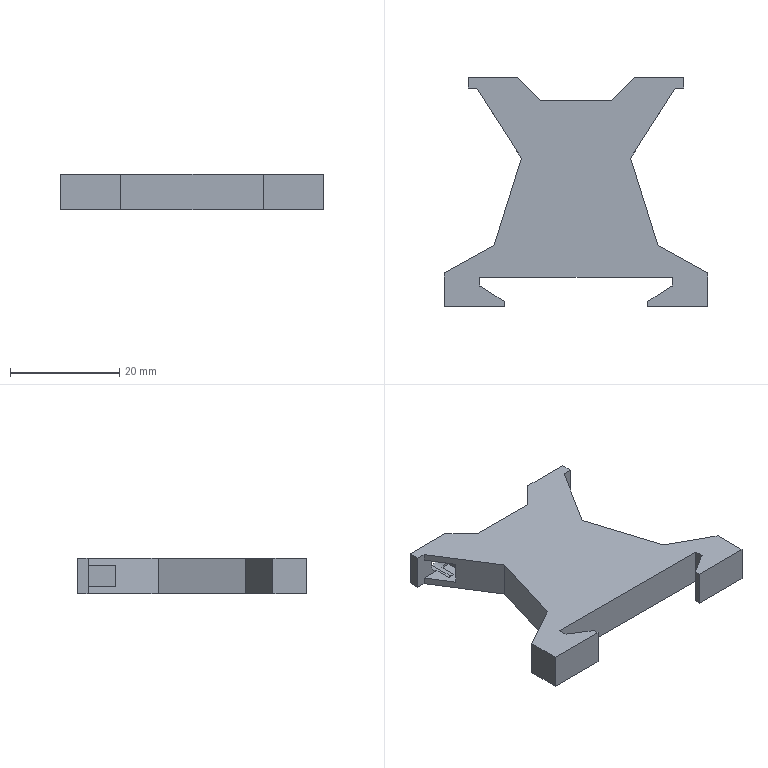Component | SolidWorks | UK5NVoltageTerminalBlock-12 | 1 solid | 48 faces | volume 6853 mm3 | plane 44 | cylinder 4 | commonest cylinder face diameters 4.2 x4